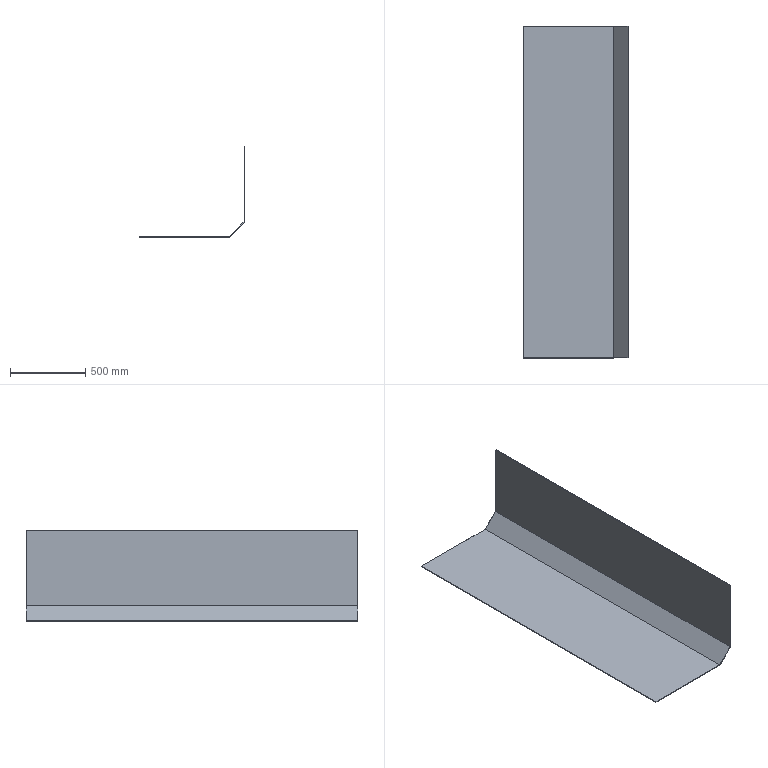Component | NX | CACAMBA_2200 | 1 solid | 10 faces | box 700 x 2200 x 600 mm | volume 13610071 mm3 | plane 10
STEP:
#1=CARTESIAN_POINT('',(0.,0.,0.));
#2=DIRECTION('',(0.,0.,1.));
#3=DIRECTION('',(1.,0.,0.));
#4=AXIS2_PLACEMENT_3D('',#1,#2,#3);
#5=CARTESIAN_POINT('',(-10.,765.233,680.));
#6=VERTEX_POINT('',#5);
#7=CARTESIAN_POINT('',(-10.,765.233,180.));
#8=VERTEX_POINT('',#7);
#9=CARTESIAN_POINT('',(-10.,765.233,680.));
#10=DIRECTION('',(0.,0.,-1.));
#11=VECTOR('',#10,1.);
#12=LINE('',#9,#11);
#13=CARTESIAN_POINT('',(-10.,-1434.767,680.));
#14=DIRECTION('',(1.,0.,0.));
#15=DIRECTION('',(0.,0.,1.));
#16=AXIS2_PLACEMENT_3D('',#13,#14,#15);
#17=PLANE('',#16);
#18=CARTESIAN_POINT('',(0.,-2200.));
#19=DIRECTION('',(-1.,0.));
#20=VECTOR('',#19,1.);
#21=LINE('',#18,#20);
#22=(GEOMETRIC_REPRESENTATION_CONTEXT(2)PARAMETRIC_REPRESENTATION_CONTEXT()REPRESENTATION_CONTEXT('',''));
#23=DEFINITIONAL_REPRESENTATION('',(#21),#22);
#24=PCURVE('',#17,#23);
#25=CARTESIAN_POINT('',(-10.,765.233,80.));
#26=DIRECTION('',(0.,1.,0.));
#27=DIRECTION('',(0.,0.,-1.));
#28=AXIS2_PLACEMENT_3D('',#25,#26,#27);
#29=PLANE('',#28);
#30=CARTESIAN_POINT('',(-600.,0.));
#31=DIRECTION('',(1.,0.));
#32=VECTOR('',#31,1.);
#33=LINE('',#30,#32);
#34=(GEOMETRIC_REPRESENTATION_CONTEXT(2)PARAMETRIC_REPRESENTATION_CONTEXT()REPRESENTATION_CONTEXT('',''));
#35=DEFINITIONAL_REPRESENTATION('',(#33),#34);
#36=PCURVE('',#29,#35);
#37=SURFACE_CURVE('',#12,(#24,#36),.PCURVE_S1.);
#38=EDGE_CURVE('',#6,#8,#37,.T.);
#39=ORIENTED_EDGE('',*,*,#38,.F.);
#40=CARTESIAN_POINT('',(-10.,-1434.767,680.));
#41=VERTEX_POINT('',#40);
#42=CARTESIAN_POINT('',(-10.,-1434.767,680.));
#43=DIRECTION('',(0.,1.,0.));
#44=VECTOR('',#43,1.);
#45=LINE('',#42,#44);
#46=CARTESIAN_POINT('',(0.,0.));
#47=DIRECTION('',(0.,-1.));
#48=VECTOR('',#47,1.);
#49=LINE('',#46,#48);
#50=(GEOMETRIC_REPRESENTATION_CONTEXT(2)PARAMETRIC_REPRESENTATION_CONTEXT()REPRESENTATION_CONTEXT('',''));
#51=DEFINITIONAL_REPRESENTATION('',(#49),#50);
#52=PCURVE('',#17,#51);
#53=CARTESIAN_POINT('',(-15.,-1434.767,680.));
#54=DIRECTION('',(0.,0.,1.));
#55=DIRECTION('',(-1.,0.,0.));
#56=AXIS2_PLACEMENT_3D('',#53,#54,#55);
#57=PLANE('',#56);
#58=CARTESIAN_POINT('',(-5.,0.));
#59=DIRECTION('',(0.,-1.));
#60=VECTOR('',#59,1.);
#61=LINE('',#58,#60);
#62=(GEOMETRIC_REPRESENTATION_CONTEXT(2)PARAMETRIC_REPRESENTATION_CONTEXT()REPRESENTATION_CONTEXT('',''));
#63=DEFINITIONAL_REPRESENTATION('',(#61),#62);
#64=PCURVE('',#57,#63);
#65=SURFACE_CURVE('',#45,(#52,#64),.PCURVE_S1.);
#66=EDGE_CURVE('',#41,#6,#65,.T.);
#67=ORIENTED_EDGE('',*,*,#66,.F.);
#68=CARTESIAN_POINT('',(-10.,-1434.767,180.));
#69=VERTEX_POINT('',#68);
#70=CARTESIAN_POINT('',(-10.,-1434.767,680.));
#71=DIRECTION('',(0.,0.,-1.));
#72=VECTOR('',#71,1.);
#73=LINE('',#70,#72);
#74=CARTESIAN_POINT('',(0.,0.));
#75=DIRECTION('',(-1.,0.));
#76=VECTOR('',#75,1.);
#77=LINE('',#74,#76);
#78=(GEOMETRIC_REPRESENTATION_CONTEXT(2)PARAMETRIC_REPRESENTATION_CONTEXT()REPRESENTATION_CONTEXT('',''));
#79=DEFINITIONAL_REPRESENTATION('',(#77),#78);
#80=PCURVE('',#17,#79);
#81=CARTESIAN_POINT('',(-10.,-1434.767,80.));
#82=DIRECTION('',(0.,1.,0.));
#83=DIRECTION('',(0.,0.,-1.));
#84=AXIS2_PLACEMENT_3D('',#81,#82,#83);
#85=PLANE('',#84);
#86=CARTESIAN_POINT('',(-600.,0.));
#87=DIRECTION('',(1.,0.));
#88=VECTOR('',#87,1.);
#89=LINE('',#86,#88);
#90=(GEOMETRIC_REPRESENTATION_CONTEXT(2)PARAMETRIC_REPRESENTATION_CONTEXT()REPRESENTATION_CONTEXT('',''));
#91=DEFINITIONAL_REPRESENTATION('',(#89),#90);
#92=PCURVE('',#85,#91);
#93=SURFACE_CURVE('',#73,(#80,#92),.PCURVE_S1.);
#94=EDGE_CURVE('',#41,#69,#93,.T.);
#95=ORIENTED_EDGE('',*,*,#94,.T.);
#96=CARTESIAN_POINT('',(-10.,-1434.767,180.));
#97=DIRECTION('',(0.,1.,0.));
#98=VECTOR('',#97,1.);
#99=LINE('',#96,#98);
#100=CARTESIAN_POINT('',(-500.,0.));
#101=DIRECTION('',(0.,-1.));
#102=VECTOR('',#101,1.);
#103=LINE('',#100,#102);
#104=(GEOMETRIC_REPRESENTATION_CONTEXT(2)PARAMETRIC_REPRESENTATION_CONTEXT()REPRESENTATION_CONTEXT('',''));
#105=DEFINITIONAL_REPRESENTATION('',(#103),#104);
#106=PCURVE('',#17,#105);
#107=CARTESIAN_POINT('',(-10.,-1434.767,180.));
#108=DIRECTION('',(0.7071,0.,-0.7071));
#109=DIRECTION('',(0.7071,0.,0.7071));
#110=AXIS2_PLACEMENT_3D('',#107,#108,#109);
#111=PLANE('',#110);
#112=CARTESIAN_POINT('',(0.,0.));
#113=DIRECTION('',(0.,-1.));
#114=VECTOR('',#113,1.);
#115=LINE('',#112,#114);
#116=(GEOMETRIC_REPRESENTATION_CONTEXT(2)PARAMETRIC_REPRESENTATION_CONTEXT()REPRESENTATION_CONTEXT('',''));
#117=DEFINITIONAL_REPRESENTATION('',(#115),#116);
#118=PCURVE('',#111,#117);
#119=SURFACE_CURVE('',#99,(#106,#118),.PCURVE_S1.);
#120=EDGE_CURVE('',#69,#8,#119,.T.);
#121=ORIENTED_EDGE('',*,*,#120,.T.);
#122=EDGE_LOOP('',(#39,#67,#95,#121));
#123=FACE_BOUND('',#122,.T.);
#124=ADVANCED_FACE('',(#123),#17,.T.);
#125=CARTESIAN_POINT('',(-110.,765.233,80.));
#126=VERTEX_POINT('',#125);
#127=CARTESIAN_POINT('',(-10.,765.233,180.));
#128=DIRECTION('',(-0.7071,0.,-0.7071));
#129=VECTOR('',#128,1.);
#130=LINE('',#127,#129);
#131=CARTESIAN_POINT('',(0.,-2200.));
#132=DIRECTION('',(-1.,0.));
#133=VECTOR('',#132,1.);
#134=LINE('',#131,#133);
#135=(GEOMETRIC_REPRESENTATION_CONTEXT(2)PARAMETRIC_REPRESENTATION_CONTEXT()REPRESENTATION_CONTEXT('',''));
#136=DEFINITIONAL_REPRESENTATION('',(#134),#135);
#137=PCURVE('',#111,#136);
#138=CARTESIAN_POINT('',(-100.,0.));
#139=DIRECTION('',(0.7071,0.7071));
#140=VECTOR('',#139,1.);
#141=LINE('',#138,#140);
#142=(GEOMETRIC_REPRESENTATION_CONTEXT(2)PARAMETRIC_REPRESENTATION_CONTEXT()REPRESENTATION_CONTEXT('',''));
#143=DEFINITIONAL_REPRESENTATION('',(#141),#142);
#144=PCURVE('',#29,#143);
#145=SURFACE_CURVE('',#130,(#137,#144),.PCURVE_S1.);
#146=EDGE_CURVE('',#8,#126,#145,.T.);
#147=ORIENTED_EDGE('',*,*,#146,.F.);
#148=ORIENTED_EDGE('',*,*,#120,.F.);
#149=CARTESIAN_POINT('',(-110.,-1434.767,80.));
#150=VERTEX_POINT('',#149);
#151=CARTESIAN_POINT('',(-10.,-1434.767,180.));
#152=DIRECTION('',(-0.7071,0.,-0.7071));
#153=VECTOR('',#152,1.);
#154=LINE('',#151,#153);
#155=CARTESIAN_POINT('',(0.,0.));
#156=DIRECTION('',(-1.,0.));
#157=VECTOR('',#156,1.);
#158=LINE('',#155,#157);
#159=(GEOMETRIC_REPRESENTATION_CONTEXT(2)PARAMETRIC_REPRESENTATION_CONTEXT()REPRESENTATION_CONTEXT('',''));
#160=DEFINITIONAL_REPRESENTATION('',(#158),#159);
#161=PCURVE('',#111,#160);
#162=CARTESIAN_POINT('',(-100.,0.));
#163=DIRECTION('',(0.7071,0.7071));
#164=VECTOR('',#163,1.);
#165=LINE('',#162,#164);
#166=(GEOMETRIC_REPRESENTATION_CONTEXT(2)PARAMETRIC_REPRESENTATION_CONTEXT()REPRESENTATION_CONTEXT('',''));
#167=DEFINITIONAL_REPRESENTATION('',(#165),#166);
#168=PCURVE('',#85,#167);
#169=SURFACE_CURVE('',#154,(#161,#168),.PCURVE_S1.);
#170=EDGE_CURVE('',#69,#150,#169,.T.);
#171=ORIENTED_EDGE('',*,*,#170,.T.);
#172=CARTESIAN_POINT('',(-110.,-1434.767,80.));
#173=DIRECTION('',(0.,1.,0.));
#174=VECTOR('',#173,1.);
#175=LINE('',#172,#174);
#176=CARTESIAN_POINT('',(-141.421,0.));
#177=DIRECTION('',(0.,-1.));
#178=VECTOR('',#177,1.);
#179=LINE('',#176,#178);
#180=(GEOMETRIC_REPRESENTATION_CONTEXT(2)PARAMETRIC_REPRESENTATION_CONTEXT()REPRESENTATION_CONTEXT('',''));
#181=DEFINITIONAL_REPRESENTATION('',(#179),#180);
#182=PCURVE('',#111,#181);
#183=CARTESIAN_POINT('',(-110.,-1434.767,80.));
#184=DIRECTION('',(0.,0.,-1.));
#185=DIRECTION('',(1.,0.,0.));
#186=AXIS2_PLACEMENT_3D('',#183,#184,#185);
#187=PLANE('',#186);
#188=CARTESIAN_POINT('',(0.,0.));
#189=DIRECTION('',(0.,-1.));
#190=VECTOR('',#189,1.);
#191=LINE('',#188,#190);
#192=(GEOMETRIC_REPRESENTATION_CONTEXT(2)PARAMETRIC_REPRESENTATION_CONTEXT()REPRESENTATION_CONTEXT('',''));
#193=DEFINITIONAL_REPRESENTATION('',(#191),#192);
#194=PCURVE('',#187,#193);
#195=SURFACE_CURVE('',#175,(#182,#194),.PCURVE_S1.);
#196=EDGE_CURVE('',#150,#126,#195,.T.);
#197=ORIENTED_EDGE('',*,*,#196,.T.);
#198=EDGE_LOOP('',(#147,#148,#171,#197));
#199=FACE_BOUND('',#198,.T.);
#200=ADVANCED_FACE('',(#199),#111,.T.);
#201=CARTESIAN_POINT('',(-710.,765.233,80.));
#202=VERTEX_POINT('',#201);
#203=CARTESIAN_POINT('',(-110.,765.233,80.));
#204=DIRECTION('',(-1.,0.,0.));
#205=VECTOR('',#204,1.);
#206=LINE('',#203,#205);
#207=CARTESIAN_POINT('',(0.,-2200.));
#208=DIRECTION('',(-1.,0.));
#209=VECTOR('',#208,1.);
#210=LINE('',#207,#209);
#211=(GEOMETRIC_REPRESENTATION_CONTEXT(2)PARAMETRIC_REPRESENTATION_CONTEXT()REPRESENTATION_CONTEXT('',''));
#212=DEFINITIONAL_REPRESENTATION('',(#210),#211);
#213=PCURVE('',#187,#212);
#214=CARTESIAN_POINT('',(0.,100.));
#215=DIRECTION('',(0.,1.));
#216=VECTOR('',#215,1.);
#217=LINE('',#214,#216);
#218=(GEOMETRIC_REPRESENTATION_CONTEXT(2)PARAMETRIC_REPRESENTATION_CONTEXT()REPRESENTATION_CONTEXT('',''));
#219=DEFINITIONAL_REPRESENTATION('',(#217),#218);
#220=PCURVE('',#29,#219);
#221=SURFACE_CURVE('',#206,(#213,#220),.PCURVE_S1.);
#222=EDGE_CURVE('',#126,#202,#221,.T.);
#223=ORIENTED_EDGE('',*,*,#222,.F.);
#224=ORIENTED_EDGE('',*,*,#196,.F.);
#225=CARTESIAN_POINT('',(-710.,-1434.767,80.));
#226=VERTEX_POINT('',#225);
#227=CARTESIAN_POINT('',(-110.,-1434.767,80.));
#228=DIRECTION('',(-1.,0.,0.));
#229=VECTOR('',#228,1.);
#230=LINE('',#227,#229);
#231=CARTESIAN_POINT('',(0.,0.));
#232=DIRECTION('',(-1.,0.));
#233=VECTOR('',#232,1.);
#234=LINE('',#231,#233);
#235=(GEOMETRIC_REPRESENTATION_CONTEXT(2)PARAMETRIC_REPRESENTATION_CONTEXT()REPRESENTATION_CONTEXT('',''));
#236=DEFINITIONAL_REPRESENTATION('',(#234),#235);
#237=PCURVE('',#187,#236);
#238=CARTESIAN_POINT('',(0.,100.));
#239=DIRECTION('',(0.,1.));
#240=VECTOR('',#239,1.);
#241=LINE('',#238,#240);
#242=(GEOMETRIC_REPRESENTATION_CONTEXT(2)PARAMETRIC_REPRESENTATION_CONTEXT()REPRESENTATION_CONTEXT('',''));
#243=DEFINITIONAL_REPRESENTATION('',(#241),#242);
#244=PCURVE('',#85,#243);
#245=SURFACE_CURVE('',#230,(#237,#244),.PCURVE_S1.);
#246=EDGE_CURVE('',#150,#226,#245,.T.);
#247=ORIENTED_EDGE('',*,*,#246,.T.);
#248=CARTESIAN_POINT('',(-710.,-1434.767,80.));
#249=DIRECTION('',(0.,1.,0.));
#250=VECTOR('',#249,1.);
#251=LINE('',#248,#250);
#252=CARTESIAN_POINT('',(-600.,0.));
#253=DIRECTION('',(0.,-1.));
#254=VECTOR('',#253,1.);
#255=LINE('',#252,#254);
#256=(GEOMETRIC_REPRESENTATION_CONTEXT(2)PARAMETRIC_REPRESENTATION_CONTEXT()REPRESENTATION_CONTEXT('',''));
#257=DEFINITIONAL_REPRESENTATION('',(#255),#256);
#258=PCURVE('',#187,#257);
#259=CARTESIAN_POINT('',(-710.,-1434.767,80.));
#260=DIRECTION('',(-1.,0.,0.));
#261=DIRECTION('',(0.,0.,-1.));
#262=AXIS2_PLACEMENT_3D('',#259,#260,#261);
#263=PLANE('',#262);
#264=CARTESIAN_POINT('',(0.,0.));
#265=DIRECTION('',(0.,-1.));
#266=VECTOR('',#265,1.);
#267=LINE('',#264,#266);
#268=(GEOMETRIC_REPRESENTATION_CONTEXT(2)PARAMETRIC_REPRESENTATION_CONTEXT()REPRESENTATION_CONTEXT('',''));
#269=DEFINITIONAL_REPRESENTATION('',(#267),#268);
#270=PCURVE('',#263,#269);
#271=SURFACE_CURVE('',#251,(#258,#270),.PCURVE_S1.);
#272=EDGE_CURVE('',#226,#202,#271,.T.);
#273=ORIENTED_EDGE('',*,*,#272,.T.);
#274=EDGE_LOOP('',(#223,#224,#247,#273));
#275=FACE_BOUND('',#274,.T.);
#276=ADVANCED_FACE('',(#275),#187,.T.);
#277=CARTESIAN_POINT('',(-710.,765.233,85.));
#278=VERTEX_POINT('',#277);
#279=CARTESIAN_POINT('',(-710.,765.233,80.));
#280=DIRECTION('',(0.,0.,1.));
#281=VECTOR('',#280,1.);
#282=LINE('',#279,#281);
#283=CARTESIAN_POINT('',(0.,-2200.));
#284=DIRECTION('',(-1.,0.));
#285=VECTOR('',#284,1.);
#286=LINE('',#283,#285);
#287=(GEOMETRIC_REPRESENTATION_CONTEXT(2)PARAMETRIC_REPRESENTATION_CONTEXT()REPRESENTATION_CONTEXT('',''));
#288=DEFINITIONAL_REPRESENTATION('',(#286),#287);
#289=PCURVE('',#263,#288);
#290=CARTESIAN_POINT('',(0.,700.));
#291=DIRECTION('',(-1.,0.));
#292=VECTOR('',#291,1.);
#293=LINE('',#290,#292);
#294=(GEOMETRIC_REPRESENTATION_CONTEXT(2)PARAMETRIC_REPRESENTATION_CONTEXT()REPRESENTATION_CONTEXT('',''));
#295=DEFINITIONAL_REPRESENTATION('',(#293),#294);
#296=PCURVE('',#29,#295);
#297=SURFACE_CURVE('',#282,(#289,#296),.PCURVE_S1.);
#298=EDGE_CURVE('',#202,#278,#297,.T.);
#299=ORIENTED_EDGE('',*,*,#298,.F.);
#300=ORIENTED_EDGE('',*,*,#272,.F.);
#301=CARTESIAN_POINT('',(-710.,-1434.767,85.));
#302=VERTEX_POINT('',#301);
#303=CARTESIAN_POINT('',(-710.,-1434.767,80.));
#304=DIRECTION('',(0.,0.,1.));
#305=VECTOR('',#304,1.);
#306=LINE('',#303,#305);
#307=CARTESIAN_POINT('',(0.,0.));
#308=DIRECTION('',(-1.,0.));
#309=VECTOR('',#308,1.);
#310=LINE('',#307,#309);
#311=(GEOMETRIC_REPRESENTATION_CONTEXT(2)PARAMETRIC_REPRESENTATION_CONTEXT()REPRESENTATION_CONTEXT('',''));
#312=DEFINITIONAL_REPRESENTATION('',(#310),#311);
#313=PCURVE('',#263,#312);
#314=CARTESIAN_POINT('',(0.,700.));
#315=DIRECTION('',(-1.,0.));
#316=VECTOR('',#315,1.);
#317=LINE('',#314,#316);
#318=(GEOMETRIC_REPRESENTATION_CONTEXT(2)PARAMETRIC_REPRESENTATION_CONTEXT()REPRESENTATION_CONTEXT('',''));
#319=DEFINITIONAL_REPRESENTATION('',(#317),#318);
#320=PCURVE('',#85,#319);
#321=SURFACE_CURVE('',#306,(#313,#320),.PCURVE_S1.);
#322=EDGE_CURVE('',#226,#302,#321,.T.);
#323=ORIENTED_EDGE('',*,*,#322,.T.);
#324=CARTESIAN_POINT('',(-710.,-1434.767,85.));
#325=DIRECTION('',(0.,1.,0.));
#326=VECTOR('',#325,1.);
#327=LINE('',#324,#326);
#328=CARTESIAN_POINT('',(-5.,0.));
#329=DIRECTION('',(0.,-1.));
#330=VECTOR('',#329,1.);
#331=LINE('',#328,#330);
#332=(GEOMETRIC_REPRESENTATION_CONTEXT(2)PARAMETRIC_REPRESENTATION_CONTEXT()REPRESENTATION_CONTEXT('',''));
#333=DEFINITIONAL_REPRESENTATION('',(#331),#332);
#334=PCURVE('',#263,#333);
#335=CARTESIAN_POINT('',(-710.,-1434.767,85.));
#336=DIRECTION('',(0.,0.,1.));
#337=DIRECTION('',(-1.,0.,0.));
#338=AXIS2_PLACEMENT_3D('',#335,#336,#337);
#339=PLANE('',#338);
#340=CARTESIAN_POINT('',(0.,0.));
#341=DIRECTION('',(0.,-1.));
#342=VECTOR('',#341,1.);
#343=LINE('',#340,#342);
#344=(GEOMETRIC_REPRESENTATION_CONTEXT(2)PARAMETRIC_REPRESENTATION_CONTEXT()REPRESENTATION_CONTEXT('',''));
#345=DEFINITIONAL_REPRESENTATION('',(#343),#344);
#346=PCURVE('',#339,#345);
#347=SURFACE_CURVE('',#327,(#334,#346),.PCURVE_S1.);
#348=EDGE_CURVE('',#302,#278,#347,.T.);
#349=ORIENTED_EDGE('',*,*,#348,.T.);
#350=EDGE_LOOP('',(#299,#300,#323,#349));
#351=FACE_BOUND('',#350,.T.);
#352=ADVANCED_FACE('',(#351),#263,.T.);
#353=CARTESIAN_POINT('',(-112.071,765.233,85.));
#354=VERTEX_POINT('',#353);
#355=CARTESIAN_POINT('',(-710.,765.233,85.));
#356=DIRECTION('',(1.,0.,0.));
#357=VECTOR('',#356,1.);
#358=LINE('',#355,#357);
#359=CARTESIAN_POINT('',(0.,-2200.));
#360=DIRECTION('',(-1.,0.));
#361=VECTOR('',#360,1.);
#362=LINE('',#359,#361);
#363=(GEOMETRIC_REPRESENTATION_CONTEXT(2)PARAMETRIC_REPRESENTATION_CONTEXT()REPRESENTATION_CONTEXT('',''));
#364=DEFINITIONAL_REPRESENTATION('',(#362),#363);
#365=PCURVE('',#339,#364);
#366=CARTESIAN_POINT('',(-5.,700.));
#367=DIRECTION('',(0.,-1.));
#368=VECTOR('',#367,1.);
#369=LINE('',#366,#368);
#370=(GEOMETRIC_REPRESENTATION_CONTEXT(2)PARAMETRIC_REPRESENTATION_CONTEXT()REPRESENTATION_CONTEXT('',''));
#371=DEFINITIONAL_REPRESENTATION('',(#369),#370);
#372=PCURVE('',#29,#371);
#373=SURFACE_CURVE('',#358,(#365,#372),.PCURVE_S1.);
#374=EDGE_CURVE('',#278,#354,#373,.T.);
#375=ORIENTED_EDGE('',*,*,#374,.F.);
#376=ORIENTED_EDGE('',*,*,#348,.F.);
#377=CARTESIAN_POINT('',(-112.071,-1434.767,85.));
#378=VERTEX_POINT('',#377);
#379=CARTESIAN_POINT('',(-710.,-1434.767,85.));
#380=DIRECTION('',(1.,0.,0.));
#381=VECTOR('',#380,1.);
#382=LINE('',#379,#381);
#383=CARTESIAN_POINT('',(0.,0.));
#384=DIRECTION('',(-1.,0.));
#385=VECTOR('',#384,1.);
#386=LINE('',#383,#385);
#387=(GEOMETRIC_REPRESENTATION_CONTEXT(2)PARAMETRIC_REPRESENTATION_CONTEXT()REPRESENTATION_CONTEXT('',''));
#388=DEFINITIONAL_REPRESENTATION('',(#386),#387);
#389=PCURVE('',#339,#388);
#390=CARTESIAN_POINT('',(-5.,700.));
#391=DIRECTION('',(0.,-1.));
#392=VECTOR('',#391,1.);
#393=LINE('',#390,#392);
#394=(GEOMETRIC_REPRESENTATION_CONTEXT(2)PARAMETRIC_REPRESENTATION_CONTEXT()REPRESENTATION_CONTEXT('',''));
#395=DEFINITIONAL_REPRESENTATION('',(#393),#394);
#396=PCURVE('',#85,#395);
#397=SURFACE_CURVE('',#382,(#389,#396),.PCURVE_S1.);
#398=EDGE_CURVE('',#302,#378,#397,.T.);
#399=ORIENTED_EDGE('',*,*,#398,.T.);
#400=CARTESIAN_POINT('',(-112.071,-1434.767,85.));
#401=DIRECTION('',(0.,1.,0.));
#402=VECTOR('',#401,1.);
#403=LINE('',#400,#402);
#404=CARTESIAN_POINT('',(-597.929,0.));
#405=DIRECTION('',(0.,-1.));
#406=VECTOR('',#405,1.);
#407=LINE('',#404,#406);
#408=(GEOMETRIC_REPRESENTATION_CONTEXT(2)PARAMETRIC_REPRESENTATION_CONTEXT()REPRESENTATION_CONTEXT('',''));
#409=DEFINITIONAL_REPRESENTATION('',(#407),#408);
#410=PCURVE('',#339,#409);
#411=CARTESIAN_POINT('',(-112.071,-1434.767,85.));
#412=DIRECTION('',(-0.7071,0.,0.7071));
#413=DIRECTION('',(-0.7071,0.,-0.7071));
#414=AXIS2_PLACEMENT_3D('',#411,#412,#413);
#415=PLANE('',#414);
#416=CARTESIAN_POINT('',(0.,0.));
#417=DIRECTION('',(0.,-1.));
#418=VECTOR('',#417,1.);
#419=LINE('',#416,#418);
#420=(GEOMETRIC_REPRESENTATION_CONTEXT(2)PARAMETRIC_REPRESENTATION_CONTEXT()REPRESENTATION_CONTEXT('',''));
#421=DEFINITIONAL_REPRESENTATION('',(#419),#420);
#422=PCURVE('',#415,#421);
#423=SURFACE_CURVE('',#403,(#410,#422),.PCURVE_S1.);
#424=EDGE_CURVE('',#378,#354,#423,.T.);
#425=ORIENTED_EDGE('',*,*,#424,.T.);
#426=EDGE_LOOP('',(#375,#376,#399,#425));
#427=FACE_BOUND('',#426,.T.);
#428=ADVANCED_FACE('',(#427),#339,.T.);
#429=CARTESIAN_POINT('',(-15.,765.233,182.071));
#430=VERTEX_POINT('',#429);
#431=CARTESIAN_POINT('',(-112.071,765.233,85.));
#432=DIRECTION('',(0.7071,0.,0.7071));
#433=VECTOR('',#432,1.);
#434=LINE('',#431,#433);
#435=CARTESIAN_POINT('',(0.,-2200.));
#436=DIRECTION('',(-1.,0.));
#437=VECTOR('',#436,1.);
#438=LINE('',#435,#437);
#439=(GEOMETRIC_REPRESENTATION_CONTEXT(2)PARAMETRIC_REPRESENTATION_CONTEXT()REPRESENTATION_CONTEXT('',''));
#440=DEFINITIONAL_REPRESENTATION('',(#438),#439);
#441=PCURVE('',#415,#440);
#442=CARTESIAN_POINT('',(-5.,102.071));
#443=DIRECTION('',(-0.7071,-0.7071));
#444=VECTOR('',#443,1.);
#445=LINE('',#442,#444);
#446=(GEOMETRIC_REPRESENTATION_CONTEXT(2)PARAMETRIC_REPRESENTATION_CONTEXT()REPRESENTATION_CONTEXT('',''));
#447=DEFINITIONAL_REPRESENTATION('',(#445),#446);
#448=PCURVE('',#29,#447);
#449=SURFACE_CURVE('',#434,(#441,#448),.PCURVE_S1.);
#450=EDGE_CURVE('',#354,#430,#449,.T.);
#451=ORIENTED_EDGE('',*,*,#450,.F.);
#452=ORIENTED_EDGE('',*,*,#424,.F.);
#453=CARTESIAN_POINT('',(-15.,-1434.767,182.071));
#454=VERTEX_POINT('',#453);
#455=CARTESIAN_POINT('',(-112.071,-1434.767,85.));
#456=DIRECTION('',(0.7071,0.,0.7071));
#457=VECTOR('',#456,1.);
#458=LINE('',#455,#457);
#459=CARTESIAN_POINT('',(0.,0.));
#460=DIRECTION('',(-1.,0.));
#461=VECTOR('',#460,1.);
#462=LINE('',#459,#461);
#463=(GEOMETRIC_REPRESENTATION_CONTEXT(2)PARAMETRIC_REPRESENTATION_CONTEXT()REPRESENTATION_CONTEXT('',''));
#464=DEFINITIONAL_REPRESENTATION('',(#462),#463);
#465=PCURVE('',#415,#464);
#466=CARTESIAN_POINT('',(-5.,102.071));
#467=DIRECTION('',(-0.7071,-0.7071));
#468=VECTOR('',#467,1.);
#469=LINE('',#466,#468);
#470=(GEOMETRIC_REPRESENTATION_CONTEXT(2)PARAMETRIC_REPRESENTATION_CONTEXT()REPRESENTATION_CONTEXT('',''));
#471=DEFINITIONAL_REPRESENTATION('',(#469),#470);
#472=PCURVE('',#85,#471);
#473=SURFACE_CURVE('',#458,(#465,#472),.PCURVE_S1.);
#474=EDGE_CURVE('',#378,#454,#473,.T.);
#475=ORIENTED_EDGE('',*,*,#474,.T.);
#476=CARTESIAN_POINT('',(-15.,-1434.767,182.071));
#477=DIRECTION('',(0.,1.,0.));
#478=VECTOR('',#477,1.);
#479=LINE('',#476,#478);
#480=CARTESIAN_POINT('',(-137.279,0.));
#481=DIRECTION('',(0.,-1.));
#482=VECTOR('',#481,1.);
#483=LINE('',#480,#482);
#484=(GEOMETRIC_REPRESENTATION_CONTEXT(2)PARAMETRIC_REPRESENTATION_CONTEXT()REPRESENTATION_CONTEXT('',''));
#485=DEFINITIONAL_REPRESENTATION('',(#483),#484);
#486=PCURVE('',#415,#485);
#487=CARTESIAN_POINT('',(-15.,-1434.767,182.071));
#488=DIRECTION('',(-1.,0.,0.));
#489=DIRECTION('',(0.,0.,-1.));
#490=AXIS2_PLACEMENT_3D('',#487,#488,#489);
#491=PLANE('',#490);
#492=CARTESIAN_POINT('',(0.,0.));
#493=DIRECTION('',(0.,-1.));
#494=VECTOR('',#493,1.);
#495=LINE('',#492,#494);
#496=(GEOMETRIC_REPRESENTATION_CONTEXT(2)PARAMETRIC_REPRESENTATION_CONTEXT()REPRESENTATION_CONTEXT('',''));
#497=DEFINITIONAL_REPRESENTATION('',(#495),#496);
#498=PCURVE('',#491,#497);
#499=SURFACE_CURVE('',#479,(#486,#498),.PCURVE_S1.);
#500=EDGE_CURVE('',#454,#430,#499,.T.);
#501=ORIENTED_EDGE('',*,*,#500,.T.);
#502=EDGE_LOOP('',(#451,#452,#475,#501));
#503=FACE_BOUND('',#502,.T.);
#504=ADVANCED_FACE('',(#503),#415,.T.);
#505=CARTESIAN_POINT('',(-15.,765.233,680.));
#506=VERTEX_POINT('',#505);
#507=CARTESIAN_POINT('',(-15.,765.233,182.071));
#508=DIRECTION('',(0.,0.,1.));
#509=VECTOR('',#508,1.);
#510=LINE('',#507,#509);
#511=CARTESIAN_POINT('',(0.,-2200.));
#512=DIRECTION('',(-1.,0.));
#513=VECTOR('',#512,1.);
#514=LINE('',#511,#513);
#515=(GEOMETRIC_REPRESENTATION_CONTEXT(2)PARAMETRIC_REPRESENTATION_CONTEXT()REPRESENTATION_CONTEXT('',''));
#516=DEFINITIONAL_REPRESENTATION('',(#514),#515);
#517=PCURVE('',#491,#516);
#518=CARTESIAN_POINT('',(-102.071,5.));
#519=DIRECTION('',(-1.,0.));
#520=VECTOR('',#519,1.);
#521=LINE('',#518,#520);
#522=(GEOMETRIC_REPRESENTATION_CONTEXT(2)PARAMETRIC_REPRESENTATION_CONTEXT()REPRESENTATION_CONTEXT('',''));
#523=DEFINITIONAL_REPRESENTATION('',(#521),#522);
#524=PCURVE('',#29,#523);
#525=SURFACE_CURVE('',#510,(#517,#524),.PCURVE_S1.);
#526=EDGE_CURVE('',#430,#506,#525,.T.);
#527=ORIENTED_EDGE('',*,*,#526,.F.);
#528=ORIENTED_EDGE('',*,*,#500,.F.);
#529=CARTESIAN_POINT('',(-15.,-1434.767,680.));
#530=VERTEX_POINT('',#529);
#531=CARTESIAN_POINT('',(-15.,-1434.767,182.071));
#532=DIRECTION('',(0.,0.,1.));
#533=VECTOR('',#532,1.);
#534=LINE('',#531,#533);
#535=CARTESIAN_POINT('',(0.,0.));
#536=DIRECTION('',(-1.,0.));
#537=VECTOR('',#536,1.);
#538=LINE('',#535,#537);
#539=(GEOMETRIC_REPRESENTATION_CONTEXT(2)PARAMETRIC_REPRESENTATION_CONTEXT()REPRESENTATION_CONTEXT('',''));
#540=DEFINITIONAL_REPRESENTATION('',(#538),#539);
#541=PCURVE('',#491,#540);
#542=CARTESIAN_POINT('',(-102.071,5.));
#543=DIRECTION('',(-1.,0.));
#544=VECTOR('',#543,1.);
#545=LINE('',#542,#544);
#546=(GEOMETRIC_REPRESENTATION_CONTEXT(2)PARAMETRIC_REPRESENTATION_CONTEXT()REPRESENTATION_CONTEXT('',''));
#547=DEFINITIONAL_REPRESENTATION('',(#545),#546);
#548=PCURVE('',#85,#547);
#549=SURFACE_CURVE('',#534,(#541,#548),.PCURVE_S1.);
#550=EDGE_CURVE('',#454,#530,#549,.T.);
#551=ORIENTED_EDGE('',*,*,#550,.T.);
#552=CARTESIAN_POINT('',(-15.,-1434.767,680.));
#553=DIRECTION('',(0.,1.,0.));
#554=VECTOR('',#553,1.);
#555=LINE('',#552,#554);
#556=CARTESIAN_POINT('',(-497.929,0.));
#557=DIRECTION('',(0.,-1.));
#558=VECTOR('',#557,1.);
#559=LINE('',#556,#558);
#560=(GEOMETRIC_REPRESENTATION_CONTEXT(2)PARAMETRIC_REPRESENTATION_CONTEXT()REPRESENTATION_CONTEXT('',''));
#561=DEFINITIONAL_REPRESENTATION('',(#559),#560);
#562=PCURVE('',#491,#561);
#563=CARTESIAN_POINT('',(0.,0.));
#564=DIRECTION('',(0.,-1.));
#565=VECTOR('',#564,1.);
#566=LINE('',#563,#565);
#567=(GEOMETRIC_REPRESENTATION_CONTEXT(2)PARAMETRIC_REPRESENTATION_CONTEXT()REPRESENTATION_CONTEXT('',''));
#568=DEFINITIONAL_REPRESENTATION('',(#566),#567);
#569=PCURVE('',#57,#568);
#570=SURFACE_CURVE('',#555,(#562,#569),.PCURVE_S1.);
#571=EDGE_CURVE('',#530,#506,#570,.T.);
#572=ORIENTED_EDGE('',*,*,#571,.T.);
#573=EDGE_LOOP('',(#527,#528,#551,#572));
#574=FACE_BOUND('',#573,.T.);
#575=ADVANCED_FACE('',(#574),#491,.T.);
#576=CARTESIAN_POINT('',(-15.,765.233,680.));
#577=DIRECTION('',(1.,0.,0.));
#578=VECTOR('',#577,1.);
#579=LINE('',#576,#578);
#580=CARTESIAN_POINT('',(0.,-2200.));
#581=DIRECTION('',(-1.,0.));
#582=VECTOR('',#581,1.);
#583=LINE('',#580,#582);
#584=(GEOMETRIC_REPRESENTATION_CONTEXT(2)PARAMETRIC_REPRESENTATION_CONTEXT()REPRESENTATION_CONTEXT('',''));
#585=DEFINITIONAL_REPRESENTATION('',(#583),#584);
#586=PCURVE('',#57,#585);
#587=CARTESIAN_POINT('',(-600.,5.));
#588=DIRECTION('',(0.,-1.));
#589=VECTOR('',#588,1.);
#590=LINE('',#587,#589);
#591=(GEOMETRIC_REPRESENTATION_CONTEXT(2)PARAMETRIC_REPRESENTATION_CONTEXT()REPRESENTATION_CONTEXT('',''));
#592=DEFINITIONAL_REPRESENTATION('',(#590),#591);
#593=PCURVE('',#29,#592);
#594=SURFACE_CURVE('',#579,(#586,#593),.PCURVE_S1.);
#595=EDGE_CURVE('',#506,#6,#594,.T.);
#596=ORIENTED_EDGE('',*,*,#595,.F.);
#597=ORIENTED_EDGE('',*,*,#571,.F.);
#598=CARTESIAN_POINT('',(-15.,-1434.767,680.));
#599=DIRECTION('',(1.,0.,0.));
#600=VECTOR('',#599,1.);
#601=LINE('',#598,#600);
#602=CARTESIAN_POINT('',(0.,0.));
#603=DIRECTION('',(-1.,0.));
#604=VECTOR('',#603,1.);
#605=LINE('',#602,#604);
#606=(GEOMETRIC_REPRESENTATION_CONTEXT(2)PARAMETRIC_REPRESENTATION_CONTEXT()REPRESENTATION_CONTEXT('',''));
#607=DEFINITIONAL_REPRESENTATION('',(#605),#606);
#608=PCURVE('',#57,#607);
#609=CARTESIAN_POINT('',(-600.,5.));
#610=DIRECTION('',(0.,-1.));
#611=VECTOR('',#610,1.);
#612=LINE('',#609,#611);
#613=(GEOMETRIC_REPRESENTATION_CONTEXT(2)PARAMETRIC_REPRESENTATION_CONTEXT()REPRESENTATION_CONTEXT('',''));
#614=DEFINITIONAL_REPRESENTATION('',(#612),#613);
#615=PCURVE('',#85,#614);
#616=SURFACE_CURVE('',#601,(#608,#615),.PCURVE_S1.);
#617=EDGE_CURVE('',#530,#41,#616,.T.);
#618=ORIENTED_EDGE('',*,*,#617,.T.);
#619=ORIENTED_EDGE('',*,*,#66,.T.);
#620=EDGE_LOOP('',(#596,#597,#618,#619));
#621=FACE_BOUND('',#620,.T.);
#622=ADVANCED_FACE('',(#621),#57,.T.);
#623=ORIENTED_EDGE('',*,*,#94,.F.);
#624=ORIENTED_EDGE('',*,*,#617,.F.);
#625=ORIENTED_EDGE('',*,*,#550,.F.);
#626=ORIENTED_EDGE('',*,*,#474,.F.);
#627=ORIENTED_EDGE('',*,*,#398,.F.);
#628=ORIENTED_EDGE('',*,*,#322,.F.);
#629=ORIENTED_EDGE('',*,*,#246,.F.);
#630=ORIENTED_EDGE('',*,*,#170,.F.);
#631=EDGE_LOOP('',(#623,#624,#625,#626,#627,#628,#629,#630));
#632=FACE_BOUND('',#631,.T.);
#633=ADVANCED_FACE('',(#632),#85,.F.);
#634=ORIENTED_EDGE('',*,*,#38,.T.);
#635=ORIENTED_EDGE('',*,*,#146,.T.);
#636=ORIENTED_EDGE('',*,*,#222,.T.);
#637=ORIENTED_EDGE('',*,*,#298,.T.);
#638=ORIENTED_EDGE('',*,*,#374,.T.);
#639=ORIENTED_EDGE('',*,*,#450,.T.);
#640=ORIENTED_EDGE('',*,*,#526,.T.);
#641=ORIENTED_EDGE('',*,*,#595,.T.);
#642=EDGE_LOOP('',(#634,#635,#636,#637,#638,#639,#640,#641));
#643=FACE_BOUND('',#642,.T.);
#644=ADVANCED_FACE('',(#643),#29,.T.);
#645=CLOSED_SHELL('',(#124,#200,#276,#352,#428,#504,#575,#622,#633,#644));
#646=MANIFOLD_SOLID_BREP('',#645);
#647=(LENGTH_UNIT()NAMED_UNIT(*)SI_UNIT(.MILLI.,.METRE.));
#648=UNCERTAINTY_MEASURE_WITH_UNIT(LENGTH_MEASURE(0.0000001),#647,'','');
#649=(NAMED_UNIT(*)PLANE_ANGLE_UNIT()SI_UNIT($,.RADIAN.));
#650=(NAMED_UNIT(*)SI_UNIT($,.STERADIAN.)SOLID_ANGLE_UNIT());
#651=(GEOMETRIC_REPRESENTATION_CONTEXT(3)GLOBAL_UNCERTAINTY_ASSIGNED_CONTEXT((#648))GLOBAL_UNIT_ASSIGNED_CONTEXT((#647,#649,#650))REPRESENTATION_CONTEXT('',''));
#652=ADVANCED_BREP_SHAPE_REPRESENTATION('',(#4,#646),#651);